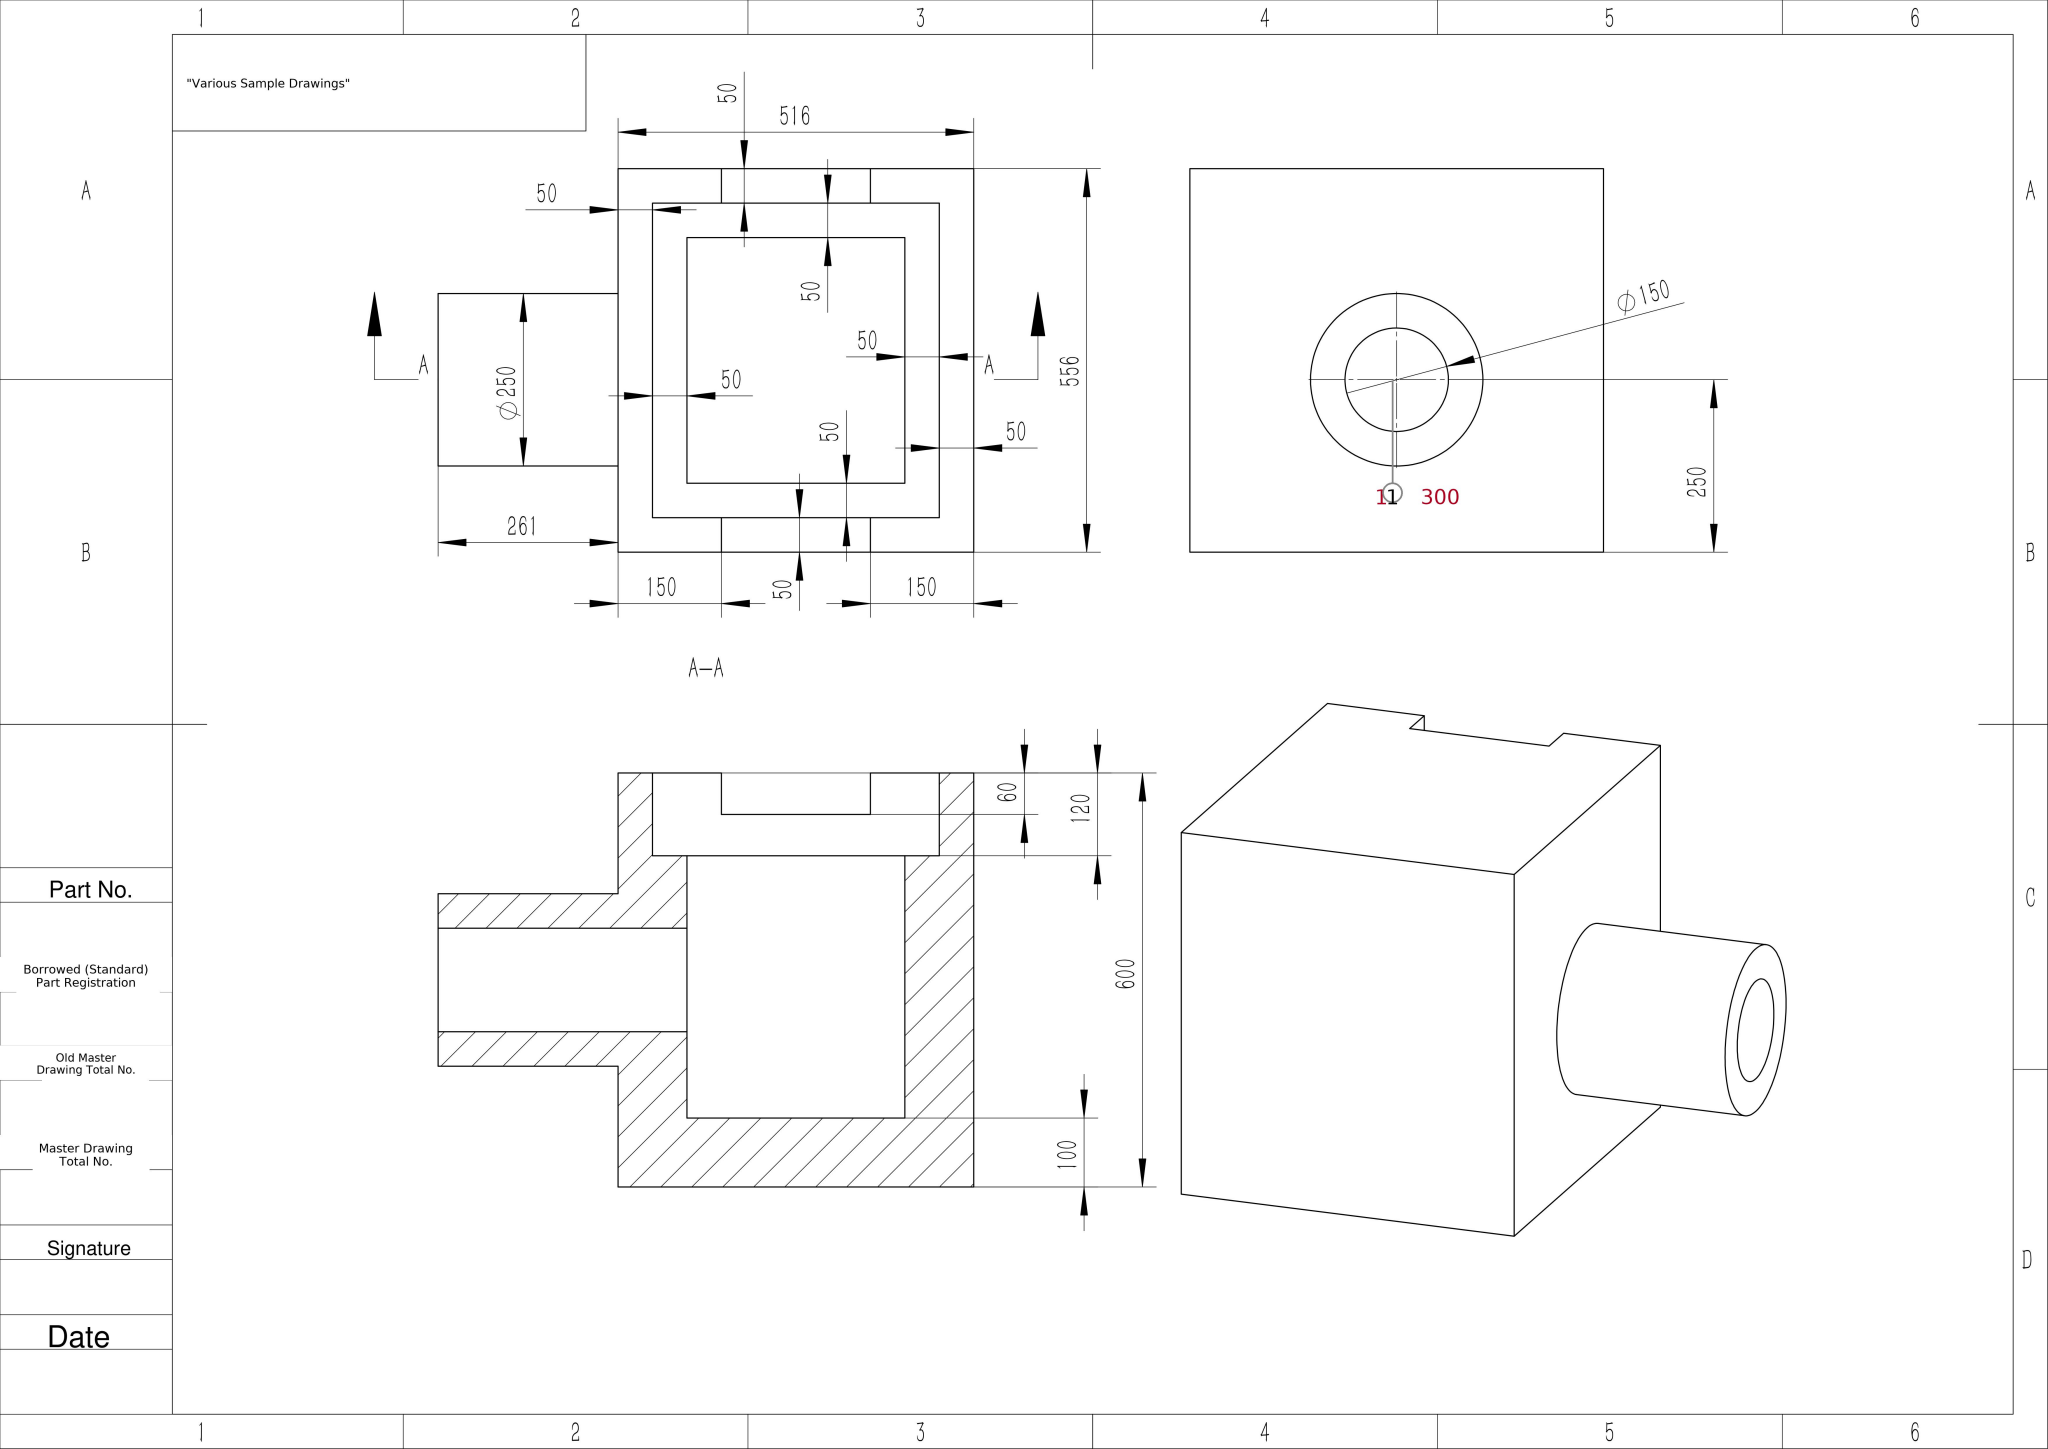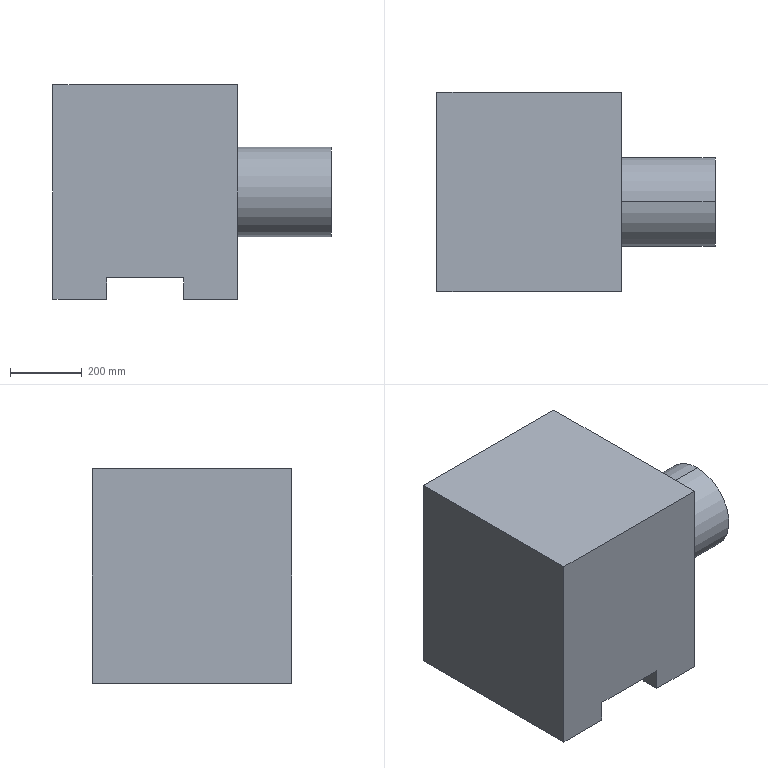Part | SolidWorks | mm | 1 solid | 28 faces | box 777 x 556 x 600 mm | volume 111762011 mm3 | plane 24 | cylinder 4 | commonest cylinder face diameters 150 x2 250 x2
build123d program:
from build123d import *

# Parameters (mm, degrees)
SKETCH1_W           = 516
SKETCH1_H           = 556
BOSS_EXTRUDE1_DEPTH = 600
SKETCH2_W           = 216
SKETCH2_H           = 597.069
CUT_EXTRUDE1_DEPTH  = 60
SKETCH3_W           = 416
SKETCH3_H           = 456
CUT_EXTRUDE2_DEPTH  = 120
SKETCH4_W           = 316
SKETCH4_H           = 356
CUT_EXTRUDE3_DEPTH  = 380
SKETCH6_R           = 125
SKETCH6_R_2         = 75
BOSS_EXTRUDE2_DEPTH = 261
CUT_EXTRUDE4_START  = -193
SKETCH7_R           = 75
CUT_EXTRUDE4_DEPTH  = 193


with BuildPart() as part:
    # Sketch1 → Boss-Extrude1 (new body)
    with BuildSketch(Plane.XY):
        Rectangle(SKETCH1_W, SKETCH1_H)
    extrude(amount=BOSS_EXTRUDE1_DEPTH)

    # Sketch2 → Cut-Extrude1 (cut)
    with BuildSketch(Plane(origin=(0, 0, 0), x_dir=(-1, 0, 0), z_dir=(0, 0, -1))):
        with Locations((0, -2.504)):
            Rectangle(SKETCH2_W, SKETCH2_H)
    extrude(amount=-CUT_EXTRUDE1_DEPTH, mode=Mode.SUBTRACT)

    # Sketch3 → Cut-Extrude2 (cut)
    with BuildSketch(Plane(origin=(0, 0, 0), x_dir=(-1, 0, 0), z_dir=(0, 0, -1))):
        Rectangle(SKETCH3_W, SKETCH3_H)
    extrude(amount=-CUT_EXTRUDE2_DEPTH, mode=Mode.SUBTRACT)

    # Sketch4 → Cut-Extrude3 (cut)
    with BuildSketch(Plane(origin=(0, 0, 120), x_dir=(-1, 0, 0), z_dir=(0, 0, -1))):
        Rectangle(SKETCH4_W, SKETCH4_H)
    extrude(amount=-CUT_EXTRUDE3_DEPTH, mode=Mode.SUBTRACT)

    # Sketch6 → Boss-Extrude2 (add)
    with BuildSketch(Plane(origin=(258, 0, 0), x_dir=(0, 0, -1), z_dir=(1, 0, 0))):
        with Locations((-300, -28)):
            Circle(SKETCH6_R)
        with Locations((-300, -28)):
            Circle(SKETCH6_R_2, mode=Mode.SUBTRACT)
    extrude(amount=BOSS_EXTRUDE2_DEPTH)

    # Sketch7 → Cut-Extrude4 (cut)
    with BuildSketch(Plane(origin=(258, 0, 0), x_dir=(0, 0, -1), z_dir=(1, 0, 0)).offset(CUT_EXTRUDE4_START)):
        with Locations((-300, -28)):
            Circle(SKETCH7_R)
    extrude(amount=CUT_EXTRUDE4_DEPTH, mode=Mode.SUBTRACT)


solid = part.part
STEP:
#1=CARTESIAN_POINT('',(519.,-28.,375.));
#2=VERTEX_POINT('',#1);
#3=CARTESIAN_POINT('',(519.,-28.,225.));
#4=VERTEX_POINT('',#3);
#5=CARTESIAN_POINT('',(519.,-28.,300.));
#6=DIRECTION('',(1.,0.,0.));
#7=DIRECTION('',(0.,0.,-1.));
#8=AXIS2_PLACEMENT_3D('',#5,#6,#7);
#9=CIRCLE('',#8,75.);
#10=EDGE_CURVE('',#2,#4,#9,.T.);
#11=ORIENTED_EDGE('',*,*,#10,.T.);
#12=CARTESIAN_POINT('',(158.,-28.,225.));
#13=VERTEX_POINT('',#12);
#14=CARTESIAN_POINT('',(519.,-28.,225.));
#15=DIRECTION('',(-1.,0.,0.));
#16=VECTOR('',#15,1000.);
#17=LINE('',#14,#16);
#18=EDGE_CURVE('',#4,#13,#17,.T.);
#19=ORIENTED_EDGE('',*,*,#18,.T.);
#20=CARTESIAN_POINT('',(158.,-28.,375.));
#21=VERTEX_POINT('',#20);
#22=CARTESIAN_POINT('',(158.,-28.,300.));
#23=DIRECTION('',(1.,0.,0.));
#24=DIRECTION('',(0.,0.,-1.));
#25=AXIS2_PLACEMENT_3D('',#22,#23,#24);
#26=CIRCLE('',#25,75.);
#27=EDGE_CURVE('',#21,#13,#26,.T.);
#28=ORIENTED_EDGE('',*,*,#27,.F.);
#29=CARTESIAN_POINT('',(519.,-28.,375.));
#30=DIRECTION('',(-1.,0.,0.));
#31=VECTOR('',#30,1000.);
#32=LINE('',#29,#31);
#33=EDGE_CURVE('',#2,#21,#32,.T.);
#34=ORIENTED_EDGE('',*,*,#33,.F.);
#35=EDGE_LOOP('',(#11,#19,#28,#34));
#36=FACE_OUTER_BOUND('',#35,.T.);
#37=CARTESIAN_POINT('',(519.,-28.,300.));
#38=DIRECTION('',(-1.,0.,0.));
#39=DIRECTION('',(0.,0.,1.));
#40=AXIS2_PLACEMENT_3D('',#37,#38,#39);
#41=CYLINDRICAL_SURFACE('',#40,75.);
#42=ADVANCED_FACE('',(#36),#41,.F.);
#43=CARTESIAN_POINT('',(519.,-28.,175.));
#44=VERTEX_POINT('',#43);
#45=CARTESIAN_POINT('',(519.,-28.,425.));
#46=VERTEX_POINT('',#45);
#47=CARTESIAN_POINT('',(519.,-28.,300.));
#48=DIRECTION('',(1.,0.,0.));
#49=DIRECTION('',(0.,0.,-1.));
#50=AXIS2_PLACEMENT_3D('',#47,#48,#49);
#51=CIRCLE('',#50,125.);
#52=EDGE_CURVE('',#44,#46,#51,.T.);
#53=ORIENTED_EDGE('',*,*,#52,.F.);
#54=CARTESIAN_POINT('',(258.,-28.,175.));
#55=VERTEX_POINT('',#54);
#56=CARTESIAN_POINT('',(519.,-28.,175.));
#57=DIRECTION('',(-1.,0.,0.));
#58=VECTOR('',#57,1000.);
#59=LINE('',#56,#58);
#60=EDGE_CURVE('',#44,#55,#59,.T.);
#61=ORIENTED_EDGE('',*,*,#60,.T.);
#62=CARTESIAN_POINT('',(258.,-28.,425.));
#63=VERTEX_POINT('',#62);
#64=CARTESIAN_POINT('',(258.,-28.,300.));
#65=DIRECTION('',(1.,0.,0.));
#66=DIRECTION('',(0.,0.,-1.));
#67=AXIS2_PLACEMENT_3D('',#64,#65,#66);
#68=CIRCLE('',#67,125.);
#69=EDGE_CURVE('',#55,#63,#68,.T.);
#70=ORIENTED_EDGE('',*,*,#69,.T.);
#71=CARTESIAN_POINT('',(519.,-28.,425.));
#72=DIRECTION('',(-1.,0.,0.));
#73=VECTOR('',#72,1000.);
#74=LINE('',#71,#73);
#75=EDGE_CURVE('',#46,#63,#74,.T.);
#76=ORIENTED_EDGE('',*,*,#75,.F.);
#77=EDGE_LOOP('',(#53,#61,#70,#76));
#78=FACE_OUTER_BOUND('',#77,.T.);
#79=CARTESIAN_POINT('',(519.,-28.,300.));
#80=DIRECTION('',(-1.,0.,0.));
#81=DIRECTION('',(0.,0.,1.));
#82=AXIS2_PLACEMENT_3D('',#79,#80,#81);
#83=CYLINDRICAL_SURFACE('',#82,125.);
#84=ADVANCED_FACE('',(#78),#83,.T.);
#85=CARTESIAN_POINT('',(-108.,228.,60.));
#86=VERTEX_POINT('',#85);
#87=CARTESIAN_POINT('',(108.,228.,60.));
#88=VERTEX_POINT('',#87);
#89=CARTESIAN_POINT('',(0.,228.,60.));
#90=DIRECTION('',(1.,0.,0.));
#91=VECTOR('',#90,1000.);
#92=LINE('',#89,#91);
#93=EDGE_CURVE('',#86,#88,#92,.T.);
#94=ORIENTED_EDGE('',*,*,#93,.F.);
#95=CARTESIAN_POINT('',(-108.,278.,60.));
#96=VERTEX_POINT('',#95);
#97=CARTESIAN_POINT('',(-108.,296.03,60.));
#98=DIRECTION('',(-0.,1.,0.));
#99=VECTOR('',#98,1000.);
#100=LINE('',#97,#99);
#101=EDGE_CURVE('',#86,#96,#100,.T.);
#102=ORIENTED_EDGE('',*,*,#101,.T.);
#103=CARTESIAN_POINT('',(108.,278.,60.));
#104=VERTEX_POINT('',#103);
#105=CARTESIAN_POINT('',(258.,278.,60.));
#106=DIRECTION('',(1.,0.,0.));
#107=VECTOR('',#106,1000.);
#108=LINE('',#105,#107);
#109=EDGE_CURVE('',#96,#104,#108,.T.);
#110=ORIENTED_EDGE('',*,*,#109,.T.);
#111=CARTESIAN_POINT('',(108.,296.03,60.));
#112=DIRECTION('',(-0.,-1.,0.));
#113=VECTOR('',#112,1000.);
#114=LINE('',#111,#113);
#115=EDGE_CURVE('',#104,#88,#114,.T.);
#116=ORIENTED_EDGE('',*,*,#115,.T.);
#117=EDGE_LOOP('',(#94,#102,#110,#116));
#118=FACE_OUTER_BOUND('',#117,.T.);
#119=CARTESIAN_POINT('',(0.,0.,60.));
#120=DIRECTION('',(0.,0.,-1.));
#121=DIRECTION('',(-1.,0.,0.));
#122=AXIS2_PLACEMENT_3D('',#119,#120,#121);
#123=PLANE('',#122);
#124=ADVANCED_FACE('',(#118),#123,.T.);
#125=CARTESIAN_POINT('',(108.,228.,0.));
#126=VERTEX_POINT('',#125);
#127=CARTESIAN_POINT('',(108.,278.,0.));
#128=VERTEX_POINT('',#127);
#129=CARTESIAN_POINT('',(108.,-0.,0.));
#130=DIRECTION('',(0.,1.,0.));
#131=VECTOR('',#130,1000.);
#132=LINE('',#129,#131);
#133=EDGE_CURVE('',#126,#128,#132,.T.);
#134=ORIENTED_EDGE('',*,*,#133,.F.);
#135=CARTESIAN_POINT('',(108.,228.,60.));
#136=DIRECTION('',(0.,0.,1.));
#137=VECTOR('',#136,1000.);
#138=LINE('',#135,#137);
#139=EDGE_CURVE('',#126,#88,#138,.T.);
#140=ORIENTED_EDGE('',*,*,#139,.T.);
#141=ORIENTED_EDGE('',*,*,#115,.F.);
#142=CARTESIAN_POINT('',(108.,278.,600.));
#143=DIRECTION('',(0.,0.,1.));
#144=VECTOR('',#143,1000.);
#145=LINE('',#142,#144);
#146=EDGE_CURVE('',#128,#104,#145,.T.);
#147=ORIENTED_EDGE('',*,*,#146,.F.);
#148=EDGE_LOOP('',(#134,#140,#141,#147));
#149=FACE_OUTER_BOUND('',#148,.T.);
#150=CARTESIAN_POINT('',(108.,296.03,60.));
#151=DIRECTION('',(1.,-0.,0.));
#152=DIRECTION('',(0.,1.,0.));
#153=AXIS2_PLACEMENT_3D('',#150,#151,#152);
#154=PLANE('',#153);
#155=ADVANCED_FACE('',(#149),#154,.F.);
#156=ORIENTED_EDGE('',*,*,#101,.F.);
#157=CARTESIAN_POINT('',(-108.,228.,0.));
#158=VERTEX_POINT('',#157);
#159=CARTESIAN_POINT('',(-108.,228.,60.));
#160=DIRECTION('',(0.,0.,-1.));
#161=VECTOR('',#160,1000.);
#162=LINE('',#159,#161);
#163=EDGE_CURVE('',#86,#158,#162,.T.);
#164=ORIENTED_EDGE('',*,*,#163,.T.);
#165=CARTESIAN_POINT('',(-108.,278.,0.));
#166=VERTEX_POINT('',#165);
#167=CARTESIAN_POINT('',(-108.,-0.,0.));
#168=DIRECTION('',(0.,-1.,0.));
#169=VECTOR('',#168,1000.);
#170=LINE('',#167,#169);
#171=EDGE_CURVE('',#166,#158,#170,.T.);
#172=ORIENTED_EDGE('',*,*,#171,.F.);
#173=CARTESIAN_POINT('',(-108.,278.,600.));
#174=DIRECTION('',(0.,0.,-1.));
#175=VECTOR('',#174,1000.);
#176=LINE('',#173,#175);
#177=EDGE_CURVE('',#96,#166,#176,.T.);
#178=ORIENTED_EDGE('',*,*,#177,.F.);
#179=EDGE_LOOP('',(#156,#164,#172,#178));
#180=FACE_OUTER_BOUND('',#179,.T.);
#181=CARTESIAN_POINT('',(-108.,296.03,60.));
#182=DIRECTION('',(-1.,-0.,0.));
#183=DIRECTION('',(0.,-1.,0.));
#184=AXIS2_PLACEMENT_3D('',#181,#182,#183);
#185=PLANE('',#184);
#186=ADVANCED_FACE('',(#180),#185,.F.);
#187=CARTESIAN_POINT('',(208.,228.,0.));
#188=VERTEX_POINT('',#187);
#189=CARTESIAN_POINT('',(208.,-228.,0.));
#190=VERTEX_POINT('',#189);
#191=CARTESIAN_POINT('',(208.,-228.,0.));
#192=DIRECTION('',(0.,-1.,0.));
#193=VECTOR('',#192,1000.);
#194=LINE('',#191,#193);
#195=EDGE_CURVE('',#188,#190,#194,.T.);
#196=ORIENTED_EDGE('',*,*,#195,.F.);
#197=CARTESIAN_POINT('',(-208.,228.,0.));
#198=DIRECTION('',(1.,0.,0.));
#199=VECTOR('',#198,1000.);
#200=LINE('',#197,#199);
#201=EDGE_CURVE('',#126,#188,#200,.T.);
#202=ORIENTED_EDGE('',*,*,#201,.F.);
#203=ORIENTED_EDGE('',*,*,#133,.T.);
#204=CARTESIAN_POINT('',(258.,278.,0.));
#205=VERTEX_POINT('',#204);
#206=CARTESIAN_POINT('',(258.,278.,0.));
#207=DIRECTION('',(-1.,-0.,0.));
#208=VECTOR('',#207,1000.);
#209=LINE('',#206,#208);
#210=EDGE_CURVE('',#205,#128,#209,.T.);
#211=ORIENTED_EDGE('',*,*,#210,.F.);
#212=CARTESIAN_POINT('',(258.,-278.,0.));
#213=VERTEX_POINT('',#212);
#214=CARTESIAN_POINT('',(258.,-278.,0.));
#215=DIRECTION('',(0.,1.,0.));
#216=VECTOR('',#215,1000.);
#217=LINE('',#214,#216);
#218=EDGE_CURVE('',#213,#205,#217,.T.);
#219=ORIENTED_EDGE('',*,*,#218,.F.);
#220=CARTESIAN_POINT('',(108.,-278.,0.));
#221=VERTEX_POINT('',#220);
#222=CARTESIAN_POINT('',(258.,-278.,0.));
#223=DIRECTION('',(1.,0.,0.));
#224=VECTOR('',#223,1000.);
#225=LINE('',#222,#224);
#226=EDGE_CURVE('',#221,#213,#225,.T.);
#227=ORIENTED_EDGE('',*,*,#226,.F.);
#228=CARTESIAN_POINT('',(108.,-228.,0.));
#229=VERTEX_POINT('',#228);
#230=CARTESIAN_POINT('',(108.,-0.,0.));
#231=DIRECTION('',(0.,1.,0.));
#232=VECTOR('',#231,1000.);
#233=LINE('',#230,#232);
#234=EDGE_CURVE('',#221,#229,#233,.T.);
#235=ORIENTED_EDGE('',*,*,#234,.T.);
#236=CARTESIAN_POINT('',(-208.,-228.,0.));
#237=DIRECTION('',(-1.,0.,0.));
#238=VECTOR('',#237,1000.);
#239=LINE('',#236,#238);
#240=EDGE_CURVE('',#190,#229,#239,.T.);
#241=ORIENTED_EDGE('',*,*,#240,.F.);
#242=EDGE_LOOP('',(#196,#202,#203,#211,#219,#227,#235,#241));
#243=FACE_OUTER_BOUND('',#242,.T.);
#244=CARTESIAN_POINT('',(0.,0.,0.));
#245=DIRECTION('',(0.,0.,1.));
#246=DIRECTION('',(1.,0.,0.));
#247=AXIS2_PLACEMENT_3D('',#244,#245,#246);
#248=PLANE('',#247);
#249=ADVANCED_FACE('',(#243),#248,.F.);
#250=CARTESIAN_POINT('',(-258.,278.,0.));
#251=VERTEX_POINT('',#250);
#252=CARTESIAN_POINT('',(-258.,-278.,0.));
#253=VERTEX_POINT('',#252);
#254=CARTESIAN_POINT('',(-258.,-278.,0.));
#255=DIRECTION('',(0.,-1.,0.));
#256=VECTOR('',#255,1000.);
#257=LINE('',#254,#256);
#258=EDGE_CURVE('',#251,#253,#257,.T.);
#259=ORIENTED_EDGE('',*,*,#258,.T.);
#260=CARTESIAN_POINT('',(-258.,-278.,600.));
#261=VERTEX_POINT('',#260);
#262=CARTESIAN_POINT('',(-258.,-278.,600.));
#263=DIRECTION('',(0.,0.,-1.));
#264=VECTOR('',#263,1000.);
#265=LINE('',#262,#264);
#266=EDGE_CURVE('',#261,#253,#265,.T.);
#267=ORIENTED_EDGE('',*,*,#266,.F.);
#268=CARTESIAN_POINT('',(-258.,278.,600.));
#269=VERTEX_POINT('',#268);
#270=CARTESIAN_POINT('',(-258.,-278.,600.));
#271=DIRECTION('',(0.,-1.,0.));
#272=VECTOR('',#271,1000.);
#273=LINE('',#270,#272);
#274=EDGE_CURVE('',#269,#261,#273,.T.);
#275=ORIENTED_EDGE('',*,*,#274,.F.);
#276=CARTESIAN_POINT('',(-258.,278.,600.));
#277=DIRECTION('',(0.,0.,-1.));
#278=VECTOR('',#277,1000.);
#279=LINE('',#276,#278);
#280=EDGE_CURVE('',#269,#251,#279,.T.);
#281=ORIENTED_EDGE('',*,*,#280,.T.);
#282=EDGE_LOOP('',(#259,#267,#275,#281));
#283=FACE_OUTER_BOUND('',#282,.T.);
#284=CARTESIAN_POINT('',(-258.,-278.,600.));
#285=DIRECTION('',(1.,0.,0.));
#286=DIRECTION('',(0.,0.,-1.));
#287=AXIS2_PLACEMENT_3D('',#284,#285,#286);
#288=PLANE('',#287);
#289=ADVANCED_FACE('',(#283),#288,.F.);
#290=CARTESIAN_POINT('',(108.,-278.,60.));
#291=VERTEX_POINT('',#290);
#292=CARTESIAN_POINT('',(-108.,-278.,60.));
#293=VERTEX_POINT('',#292);
#294=CARTESIAN_POINT('',(258.,-278.,60.));
#295=DIRECTION('',(-1.,-0.,0.));
#296=VECTOR('',#295,1000.);
#297=LINE('',#294,#296);
#298=EDGE_CURVE('',#291,#293,#297,.T.);
#299=ORIENTED_EDGE('',*,*,#298,.F.);
#300=CARTESIAN_POINT('',(108.,-278.,600.));
#301=DIRECTION('',(0.,0.,-1.));
#302=VECTOR('',#301,1000.);
#303=LINE('',#300,#302);
#304=EDGE_CURVE('',#291,#221,#303,.T.);
#305=ORIENTED_EDGE('',*,*,#304,.T.);
#306=ORIENTED_EDGE('',*,*,#226,.T.);
#307=CARTESIAN_POINT('',(258.,-278.,600.));
#308=VERTEX_POINT('',#307);
#309=CARTESIAN_POINT('',(258.,-278.,600.));
#310=DIRECTION('',(0.,0.,-1.));
#311=VECTOR('',#310,1000.);
#312=LINE('',#309,#311);
#313=EDGE_CURVE('',#308,#213,#312,.T.);
#314=ORIENTED_EDGE('',*,*,#313,.F.);
#315=CARTESIAN_POINT('',(258.,-278.,600.));
#316=DIRECTION('',(1.,0.,0.));
#317=VECTOR('',#316,1000.);
#318=LINE('',#315,#317);
#319=EDGE_CURVE('',#261,#308,#318,.T.);
#320=ORIENTED_EDGE('',*,*,#319,.F.);
#321=ORIENTED_EDGE('',*,*,#266,.T.);
#322=CARTESIAN_POINT('',(-108.,-278.,0.));
#323=VERTEX_POINT('',#322);
#324=CARTESIAN_POINT('',(258.,-278.,0.));
#325=DIRECTION('',(1.,0.,0.));
#326=VECTOR('',#325,1000.);
#327=LINE('',#324,#326);
#328=EDGE_CURVE('',#253,#323,#327,.T.);
#329=ORIENTED_EDGE('',*,*,#328,.T.);
#330=CARTESIAN_POINT('',(-108.,-278.,600.));
#331=DIRECTION('',(0.,0.,1.));
#332=VECTOR('',#331,1000.);
#333=LINE('',#330,#332);
#334=EDGE_CURVE('',#323,#293,#333,.T.);
#335=ORIENTED_EDGE('',*,*,#334,.T.);
#336=EDGE_LOOP('',(#299,#305,#306,#314,#320,#321,#329,#335));
#337=FACE_OUTER_BOUND('',#336,.T.);
#338=CARTESIAN_POINT('',(258.,-278.,600.));
#339=DIRECTION('',(-0.,1.,0.));
#340=DIRECTION('',(-1.,-0.,0.));
#341=AXIS2_PLACEMENT_3D('',#338,#339,#340);
#342=PLANE('',#341);
#343=ADVANCED_FACE('',(#337),#342,.F.);
#344=CARTESIAN_POINT('',(258.,-28.,300.));
#345=DIRECTION('',(1.,0.,0.));
#346=DIRECTION('',(0.,0.,-1.));
#347=AXIS2_PLACEMENT_3D('',#344,#345,#346);
#348=CIRCLE('',#347,125.);
#349=EDGE_CURVE('',#63,#55,#348,.T.);
#350=ORIENTED_EDGE('',*,*,#349,.F.);
#351=ORIENTED_EDGE('',*,*,#69,.F.);
#352=EDGE_LOOP('',(#350,#351));
#353=FACE_BOUND('',#352,.T.);
#354=ORIENTED_EDGE('',*,*,#218,.T.);
#355=CARTESIAN_POINT('',(258.,278.,600.));
#356=VERTEX_POINT('',#355);
#357=CARTESIAN_POINT('',(258.,278.,600.));
#358=DIRECTION('',(0.,0.,-1.));
#359=VECTOR('',#358,1000.);
#360=LINE('',#357,#359);
#361=EDGE_CURVE('',#356,#205,#360,.T.);
#362=ORIENTED_EDGE('',*,*,#361,.F.);
#363=CARTESIAN_POINT('',(258.,-278.,600.));
#364=DIRECTION('',(0.,1.,0.));
#365=VECTOR('',#364,1000.);
#366=LINE('',#363,#365);
#367=EDGE_CURVE('',#308,#356,#366,.T.);
#368=ORIENTED_EDGE('',*,*,#367,.F.);
#369=ORIENTED_EDGE('',*,*,#313,.T.);
#370=EDGE_LOOP('',(#354,#362,#368,#369));
#371=FACE_OUTER_BOUND('',#370,.T.);
#372=CARTESIAN_POINT('',(258.,-278.,600.));
#373=DIRECTION('',(-1.,0.,0.));
#374=DIRECTION('',(0.,0.,1.));
#375=AXIS2_PLACEMENT_3D('',#372,#373,#374);
#376=PLANE('',#375);
#377=ADVANCED_FACE('',(#353,#371),#376,.F.);
#378=ORIENTED_EDGE('',*,*,#210,.T.);
#379=ORIENTED_EDGE('',*,*,#146,.T.);
#380=ORIENTED_EDGE('',*,*,#109,.F.);
#381=ORIENTED_EDGE('',*,*,#177,.T.);
#382=CARTESIAN_POINT('',(258.,278.,0.));
#383=DIRECTION('',(-1.,-0.,0.));
#384=VECTOR('',#383,1000.);
#385=LINE('',#382,#384);
#386=EDGE_CURVE('',#166,#251,#385,.T.);
#387=ORIENTED_EDGE('',*,*,#386,.T.);
#388=ORIENTED_EDGE('',*,*,#280,.F.);
#389=CARTESIAN_POINT('',(258.,278.,600.));
#390=DIRECTION('',(-1.,-0.,0.));
#391=VECTOR('',#390,1000.);
#392=LINE('',#389,#391);
#393=EDGE_CURVE('',#356,#269,#392,.T.);
#394=ORIENTED_EDGE('',*,*,#393,.F.);
#395=ORIENTED_EDGE('',*,*,#361,.T.);
#396=EDGE_LOOP('',(#378,#379,#380,#381,#387,#388,#394,#395));
#397=FACE_OUTER_BOUND('',#396,.T.);
#398=CARTESIAN_POINT('',(258.,278.,600.));
#399=DIRECTION('',(0.,-1.,0.));
#400=DIRECTION('',(1.,0.,0.));
#401=AXIS2_PLACEMENT_3D('',#398,#399,#400);
#402=PLANE('',#401);
#403=ADVANCED_FACE('',(#397),#402,.F.);
#404=ORIENTED_EDGE('',*,*,#274,.T.);
#405=ORIENTED_EDGE('',*,*,#319,.T.);
#406=ORIENTED_EDGE('',*,*,#367,.T.);
#407=ORIENTED_EDGE('',*,*,#393,.T.);
#408=EDGE_LOOP('',(#404,#405,#406,#407));
#409=FACE_OUTER_BOUND('',#408,.T.);
#410=CARTESIAN_POINT('',(0.,0.,600.));
#411=DIRECTION('',(0.,0.,1.));
#412=DIRECTION('',(1.,0.,0.));
#413=AXIS2_PLACEMENT_3D('',#410,#411,#412);
#414=PLANE('',#413);
#415=ADVANCED_FACE('',(#409),#414,.T.);
#416=ORIENTED_EDGE('',*,*,#171,.T.);
#417=CARTESIAN_POINT('',(-208.,228.,0.));
#418=VERTEX_POINT('',#417);
#419=CARTESIAN_POINT('',(-208.,228.,0.));
#420=DIRECTION('',(1.,0.,0.));
#421=VECTOR('',#420,1000.);
#422=LINE('',#419,#421);
#423=EDGE_CURVE('',#418,#158,#422,.T.);
#424=ORIENTED_EDGE('',*,*,#423,.F.);
#425=CARTESIAN_POINT('',(-208.,-228.,0.));
#426=VERTEX_POINT('',#425);
#427=CARTESIAN_POINT('',(-208.,-228.,0.));
#428=DIRECTION('',(0.,1.,0.));
#429=VECTOR('',#428,1000.);
#430=LINE('',#427,#429);
#431=EDGE_CURVE('',#426,#418,#430,.T.);
#432=ORIENTED_EDGE('',*,*,#431,.F.);
#433=CARTESIAN_POINT('',(-108.,-228.,0.));
#434=VERTEX_POINT('',#433);
#435=CARTESIAN_POINT('',(-208.,-228.,0.));
#436=DIRECTION('',(-1.,0.,0.));
#437=VECTOR('',#436,1000.);
#438=LINE('',#435,#437);
#439=EDGE_CURVE('',#434,#426,#438,.T.);
#440=ORIENTED_EDGE('',*,*,#439,.F.);
#441=CARTESIAN_POINT('',(-108.,-0.,0.));
#442=DIRECTION('',(0.,-1.,0.));
#443=VECTOR('',#442,1000.);
#444=LINE('',#441,#443);
#445=EDGE_CURVE('',#434,#323,#444,.T.);
#446=ORIENTED_EDGE('',*,*,#445,.T.);
#447=ORIENTED_EDGE('',*,*,#328,.F.);
#448=ORIENTED_EDGE('',*,*,#258,.F.);
#449=ORIENTED_EDGE('',*,*,#386,.F.);
#450=EDGE_LOOP('',(#416,#424,#432,#440,#446,#447,#448,#449));
#451=FACE_OUTER_BOUND('',#450,.T.);
#452=CARTESIAN_POINT('',(0.,0.,0.));
#453=DIRECTION('',(0.,0.,1.));
#454=DIRECTION('',(1.,0.,0.));
#455=AXIS2_PLACEMENT_3D('',#452,#453,#454);
#456=PLANE('',#455);
#457=ADVANCED_FACE('',(#451),#456,.F.);
#458=CARTESIAN_POINT('',(108.,-228.,60.));
#459=VERTEX_POINT('',#458);
#460=CARTESIAN_POINT('',(-108.,-228.,60.));
#461=VERTEX_POINT('',#460);
#462=CARTESIAN_POINT('',(0.,-228.,60.));
#463=DIRECTION('',(-1.,0.,0.));
#464=VECTOR('',#463,1000.);
#465=LINE('',#462,#464);
#466=EDGE_CURVE('',#459,#461,#465,.T.);
#467=ORIENTED_EDGE('',*,*,#466,.F.);
#468=CARTESIAN_POINT('',(108.,296.03,60.));
#469=DIRECTION('',(-0.,-1.,0.));
#470=VECTOR('',#469,1000.);
#471=LINE('',#468,#470);
#472=EDGE_CURVE('',#459,#291,#471,.T.);
#473=ORIENTED_EDGE('',*,*,#472,.T.);
#474=ORIENTED_EDGE('',*,*,#298,.T.);
#475=CARTESIAN_POINT('',(-108.,296.03,60.));
#476=DIRECTION('',(-0.,1.,0.));
#477=VECTOR('',#476,1000.);
#478=LINE('',#475,#477);
#479=EDGE_CURVE('',#293,#461,#478,.T.);
#480=ORIENTED_EDGE('',*,*,#479,.T.);
#481=EDGE_LOOP('',(#467,#473,#474,#480));
#482=FACE_OUTER_BOUND('',#481,.T.);
#483=CARTESIAN_POINT('',(0.,0.,60.));
#484=DIRECTION('',(0.,0.,-1.));
#485=DIRECTION('',(-1.,0.,0.));
#486=AXIS2_PLACEMENT_3D('',#483,#484,#485);
#487=PLANE('',#486);
#488=ADVANCED_FACE('',(#482),#487,.T.);
#489=ORIENTED_EDGE('',*,*,#472,.F.);
#490=CARTESIAN_POINT('',(108.,-228.,60.));
#491=DIRECTION('',(0.,0.,-1.));
#492=VECTOR('',#491,1000.);
#493=LINE('',#490,#492);
#494=EDGE_CURVE('',#459,#229,#493,.T.);
#495=ORIENTED_EDGE('',*,*,#494,.T.);
#496=ORIENTED_EDGE('',*,*,#234,.F.);
#497=ORIENTED_EDGE('',*,*,#304,.F.);
#498=EDGE_LOOP('',(#489,#495,#496,#497));
#499=FACE_OUTER_BOUND('',#498,.T.);
#500=CARTESIAN_POINT('',(108.,296.03,60.));
#501=DIRECTION('',(1.,-0.,0.));
#502=DIRECTION('',(0.,1.,0.));
#503=AXIS2_PLACEMENT_3D('',#500,#501,#502);
#504=PLANE('',#503);
#505=ADVANCED_FACE('',(#499),#504,.F.);
#506=ORIENTED_EDGE('',*,*,#445,.F.);
#507=CARTESIAN_POINT('',(-108.,-228.,60.));
#508=DIRECTION('',(0.,0.,1.));
#509=VECTOR('',#508,1000.);
#510=LINE('',#507,#509);
#511=EDGE_CURVE('',#434,#461,#510,.T.);
#512=ORIENTED_EDGE('',*,*,#511,.T.);
#513=ORIENTED_EDGE('',*,*,#479,.F.);
#514=ORIENTED_EDGE('',*,*,#334,.F.);
#515=EDGE_LOOP('',(#506,#512,#513,#514));
#516=FACE_OUTER_BOUND('',#515,.T.);
#517=CARTESIAN_POINT('',(-108.,296.03,60.));
#518=DIRECTION('',(-1.,-0.,0.));
#519=DIRECTION('',(0.,-1.,0.));
#520=AXIS2_PLACEMENT_3D('',#517,#518,#519);
#521=PLANE('',#520);
#522=ADVANCED_FACE('',(#516),#521,.F.);
#523=ORIENTED_EDGE('',*,*,#201,.T.);
#524=CARTESIAN_POINT('',(208.,228.,120.));
#525=VERTEX_POINT('',#524);
#526=CARTESIAN_POINT('',(208.,228.,120.));
#527=DIRECTION('',(0.,0.,-1.));
#528=VECTOR('',#527,1000.);
#529=LINE('',#526,#528);
#530=EDGE_CURVE('',#525,#188,#529,.T.);
#531=ORIENTED_EDGE('',*,*,#530,.F.);
#532=CARTESIAN_POINT('',(-208.,228.,120.));
#533=VERTEX_POINT('',#532);
#534=CARTESIAN_POINT('',(-208.,228.,120.));
#535=DIRECTION('',(1.,0.,0.));
#536=VECTOR('',#535,1000.);
#537=LINE('',#534,#536);
#538=EDGE_CURVE('',#533,#525,#537,.T.);
#539=ORIENTED_EDGE('',*,*,#538,.F.);
#540=CARTESIAN_POINT('',(-208.,228.,120.));
#541=DIRECTION('',(0.,0.,-1.));
#542=VECTOR('',#541,1000.);
#543=LINE('',#540,#542);
#544=EDGE_CURVE('',#533,#418,#543,.T.);
#545=ORIENTED_EDGE('',*,*,#544,.T.);
#546=ORIENTED_EDGE('',*,*,#423,.T.);
#547=ORIENTED_EDGE('',*,*,#163,.F.);
#548=ORIENTED_EDGE('',*,*,#93,.T.);
#549=ORIENTED_EDGE('',*,*,#139,.F.);
#550=EDGE_LOOP('',(#523,#531,#539,#545,#546,#547,#548,#549));
#551=FACE_OUTER_BOUND('',#550,.T.);
#552=CARTESIAN_POINT('',(-208.,228.,120.));
#553=DIRECTION('',(0.,1.,0.));
#554=DIRECTION('',(0.,0.,1.));
#555=AXIS2_PLACEMENT_3D('',#552,#553,#554);
#556=PLANE('',#555);
#557=ADVANCED_FACE('',(#551),#556,.F.);
#558=ORIENTED_EDGE('',*,*,#466,.T.);
#559=ORIENTED_EDGE('',*,*,#511,.F.);
#560=ORIENTED_EDGE('',*,*,#439,.T.);
#561=CARTESIAN_POINT('',(-208.,-228.,120.));
#562=VERTEX_POINT('',#561);
#563=CARTESIAN_POINT('',(-208.,-228.,120.));
#564=DIRECTION('',(0.,0.,-1.));
#565=VECTOR('',#564,1000.);
#566=LINE('',#563,#565);
#567=EDGE_CURVE('',#562,#426,#566,.T.);
#568=ORIENTED_EDGE('',*,*,#567,.F.);
#569=CARTESIAN_POINT('',(208.,-228.,120.));
#570=VERTEX_POINT('',#569);
#571=CARTESIAN_POINT('',(-208.,-228.,120.));
#572=DIRECTION('',(-1.,0.,0.));
#573=VECTOR('',#572,1000.);
#574=LINE('',#571,#573);
#575=EDGE_CURVE('',#570,#562,#574,.T.);
#576=ORIENTED_EDGE('',*,*,#575,.F.);
#577=CARTESIAN_POINT('',(208.,-228.,120.));
#578=DIRECTION('',(0.,0.,-1.));
#579=VECTOR('',#578,1000.);
#580=LINE('',#577,#579);
#581=EDGE_CURVE('',#570,#190,#580,.T.);
#582=ORIENTED_EDGE('',*,*,#581,.T.);
#583=ORIENTED_EDGE('',*,*,#240,.T.);
#584=ORIENTED_EDGE('',*,*,#494,.F.);
#585=EDGE_LOOP('',(#558,#559,#560,#568,#576,#582,#583,#584));
#586=FACE_OUTER_BOUND('',#585,.T.);
#587=CARTESIAN_POINT('',(-208.,-228.,120.));
#588=DIRECTION('',(0.,-1.,0.));
#589=DIRECTION('',(0.,0.,-1.));
#590=AXIS2_PLACEMENT_3D('',#587,#588,#589);
#591=PLANE('',#590);
#592=ADVANCED_FACE('',(#586),#591,.F.);
#593=ORIENTED_EDGE('',*,*,#195,.T.);
#594=ORIENTED_EDGE('',*,*,#581,.F.);
#595=CARTESIAN_POINT('',(208.,-228.,120.));
#596=DIRECTION('',(0.,-1.,0.));
#597=VECTOR('',#596,1000.);
#598=LINE('',#595,#597);
#599=EDGE_CURVE('',#525,#570,#598,.T.);
#600=ORIENTED_EDGE('',*,*,#599,.F.);
#601=ORIENTED_EDGE('',*,*,#530,.T.);
#602=EDGE_LOOP('',(#593,#594,#600,#601));
#603=FACE_OUTER_BOUND('',#602,.T.);
#604=CARTESIAN_POINT('',(208.,-228.,120.));
#605=DIRECTION('',(1.,0.,0.));
#606=DIRECTION('',(0.,0.,-1.));
#607=AXIS2_PLACEMENT_3D('',#604,#605,#606);
#608=PLANE('',#607);
#609=ADVANCED_FACE('',(#603),#608,.F.);
#610=ORIENTED_EDGE('',*,*,#431,.T.);
#611=ORIENTED_EDGE('',*,*,#544,.F.);
#612=CARTESIAN_POINT('',(-208.,-228.,120.));
#613=DIRECTION('',(0.,1.,0.));
#614=VECTOR('',#613,1000.);
#615=LINE('',#612,#614);
#616=EDGE_CURVE('',#562,#533,#615,.T.);
#617=ORIENTED_EDGE('',*,*,#616,.F.);
#618=ORIENTED_EDGE('',*,*,#567,.T.);
#619=EDGE_LOOP('',(#610,#611,#617,#618));
#620=FACE_OUTER_BOUND('',#619,.T.);
#621=CARTESIAN_POINT('',(-208.,-228.,120.));
#622=DIRECTION('',(-1.,0.,0.));
#623=DIRECTION('',(0.,0.,1.));
#624=AXIS2_PLACEMENT_3D('',#621,#622,#623);
#625=PLANE('',#624);
#626=ADVANCED_FACE('',(#620),#625,.F.);
#627=CARTESIAN_POINT('',(-158.,178.,120.));
#628=VERTEX_POINT('',#627);
#629=CARTESIAN_POINT('',(158.,178.,120.));
#630=VERTEX_POINT('',#629);
#631=CARTESIAN_POINT('',(-158.,178.,120.));
#632=DIRECTION('',(1.,0.,0.));
#633=VECTOR('',#632,1000.);
#634=LINE('',#631,#633);
#635=EDGE_CURVE('',#628,#630,#634,.T.);
#636=ORIENTED_EDGE('',*,*,#635,.F.);
#637=CARTESIAN_POINT('',(-158.,-178.,120.));
#638=VERTEX_POINT('',#637);
#639=CARTESIAN_POINT('',(-158.,-178.,120.));
#640=DIRECTION('',(0.,1.,0.));
#641=VECTOR('',#640,1000.);
#642=LINE('',#639,#641);
#643=EDGE_CURVE('',#638,#628,#642,.T.);
#644=ORIENTED_EDGE('',*,*,#643,.F.);
#645=CARTESIAN_POINT('',(158.,-178.,120.));
#646=VERTEX_POINT('',#645);
#647=CARTESIAN_POINT('',(158.,-178.,120.));
#648=DIRECTION('',(-1.,0.,0.));
#649=VECTOR('',#648,1000.);
#650=LINE('',#647,#649);
#651=EDGE_CURVE('',#646,#638,#650,.T.);
#652=ORIENTED_EDGE('',*,*,#651,.F.);
#653=CARTESIAN_POINT('',(158.,178.,120.));
#654=DIRECTION('',(0.,-1.,0.));
#655=VECTOR('',#654,1000.);
#656=LINE('',#653,#655);
#657=EDGE_CURVE('',#630,#646,#656,.T.);
#658=ORIENTED_EDGE('',*,*,#657,.F.);
#659=EDGE_LOOP('',(#636,#644,#652,#658));
#660=FACE_BOUND('',#659,.T.);
#661=ORIENTED_EDGE('',*,*,#599,.T.);
#662=ORIENTED_EDGE('',*,*,#575,.T.);
#663=ORIENTED_EDGE('',*,*,#616,.T.);
#664=ORIENTED_EDGE('',*,*,#538,.T.);
#665=EDGE_LOOP('',(#661,#662,#663,#664));
#666=FACE_OUTER_BOUND('',#665,.T.);
#667=CARTESIAN_POINT('',(0.,0.,120.));
#668=DIRECTION('',(0.,0.,-1.));
#669=DIRECTION('',(-1.,0.,0.));
#670=AXIS2_PLACEMENT_3D('',#667,#668,#669);
#671=PLANE('',#670);
#672=ADVANCED_FACE('',(#660,#666),#671,.T.);
#673=ORIENTED_EDGE('',*,*,#635,.T.);
#674=CARTESIAN_POINT('',(158.,178.,500.));
#675=VERTEX_POINT('',#674);
#676=CARTESIAN_POINT('',(158.,178.,500.));
#677=DIRECTION('',(0.,0.,-1.));
#678=VECTOR('',#677,1000.);
#679=LINE('',#676,#678);
#680=EDGE_CURVE('',#675,#630,#679,.T.);
#681=ORIENTED_EDGE('',*,*,#680,.F.);
#682=CARTESIAN_POINT('',(-158.,178.,500.));
#683=VERTEX_POINT('',#682);
#684=CARTESIAN_POINT('',(-158.,178.,500.));
#685=DIRECTION('',(1.,0.,0.));
#686=VECTOR('',#685,1000.);
#687=LINE('',#684,#686);
#688=EDGE_CURVE('',#683,#675,#687,.T.);
#689=ORIENTED_EDGE('',*,*,#688,.F.);
#690=CARTESIAN_POINT('',(-158.,178.,500.));
#691=DIRECTION('',(0.,0.,-1.));
#692=VECTOR('',#691,1000.);
#693=LINE('',#690,#692);
#694=EDGE_CURVE('',#683,#628,#693,.T.);
#695=ORIENTED_EDGE('',*,*,#694,.T.);
#696=EDGE_LOOP('',(#673,#681,#689,#695));
#697=FACE_OUTER_BOUND('',#696,.T.);
#698=CARTESIAN_POINT('',(-158.,178.,500.));
#699=DIRECTION('',(0.,1.,0.));
#700=DIRECTION('',(0.,0.,1.));
#701=AXIS2_PLACEMENT_3D('',#698,#699,#700);
#702=PLANE('',#701);
#703=ADVANCED_FACE('',(#697),#702,.F.);
#704=ORIENTED_EDGE('',*,*,#643,.T.);
#705=ORIENTED_EDGE('',*,*,#694,.F.);
#706=CARTESIAN_POINT('',(-158.,-178.,500.));
#707=VERTEX_POINT('',#706);
#708=CARTESIAN_POINT('',(-158.,-178.,500.));
#709=DIRECTION('',(0.,1.,0.));
#710=VECTOR('',#709,1000.);
#711=LINE('',#708,#710);
#712=EDGE_CURVE('',#707,#683,#711,.T.);
#713=ORIENTED_EDGE('',*,*,#712,.F.);
#714=CARTESIAN_POINT('',(-158.,-178.,500.));
#715=DIRECTION('',(0.,0.,-1.));
#716=VECTOR('',#715,1000.);
#717=LINE('',#714,#716);
#718=EDGE_CURVE('',#707,#638,#717,.T.);
#719=ORIENTED_EDGE('',*,*,#718,.T.);
#720=EDGE_LOOP('',(#704,#705,#713,#719));
#721=FACE_OUTER_BOUND('',#720,.T.);
#722=CARTESIAN_POINT('',(-158.,-178.,500.));
#723=DIRECTION('',(-1.,0.,0.));
#724=DIRECTION('',(0.,0.,1.));
#725=AXIS2_PLACEMENT_3D('',#722,#723,#724);
#726=PLANE('',#725);
#727=ADVANCED_FACE('',(#721),#726,.F.);
#728=ORIENTED_EDGE('',*,*,#651,.T.);
#729=ORIENTED_EDGE('',*,*,#718,.F.);
#730=CARTESIAN_POINT('',(158.,-178.,500.));
#731=VERTEX_POINT('',#730);
#732=CARTESIAN_POINT('',(158.,-178.,500.));
#733=DIRECTION('',(-1.,0.,0.));
#734=VECTOR('',#733,1000.);
#735=LINE('',#732,#734);
#736=EDGE_CURVE('',#731,#707,#735,.T.);
#737=ORIENTED_EDGE('',*,*,#736,.F.);
#738=CARTESIAN_POINT('',(158.,-178.,500.));
#739=DIRECTION('',(0.,0.,-1.));
#740=VECTOR('',#739,1000.);
#741=LINE('',#738,#740);
#742=EDGE_CURVE('',#731,#646,#741,.T.);
#743=ORIENTED_EDGE('',*,*,#742,.T.);
#744=EDGE_LOOP('',(#728,#729,#737,#743));
#745=FACE_OUTER_BOUND('',#744,.T.);
#746=CARTESIAN_POINT('',(158.,-178.,500.));
#747=DIRECTION('',(0.,-1.,0.));
#748=DIRECTION('',(0.,0.,-1.));
#749=AXIS2_PLACEMENT_3D('',#746,#747,#748);
#750=PLANE('',#749);
#751=ADVANCED_FACE('',(#745),#750,.F.);
#752=ORIENTED_EDGE('',*,*,#27,.T.);
#753=CARTESIAN_POINT('',(158.,-28.,300.));
#754=DIRECTION('',(1.,0.,0.));
#755=DIRECTION('',(0.,0.,-1.));
#756=AXIS2_PLACEMENT_3D('',#753,#754,#755);
#757=CIRCLE('',#756,75.);
#758=EDGE_CURVE('',#13,#21,#757,.T.);
#759=ORIENTED_EDGE('',*,*,#758,.T.);
#760=EDGE_LOOP('',(#752,#759));
#761=FACE_BOUND('',#760,.T.);
#762=ORIENTED_EDGE('',*,*,#657,.T.);
#763=ORIENTED_EDGE('',*,*,#742,.F.);
#764=CARTESIAN_POINT('',(158.,178.,500.));
#765=DIRECTION('',(0.,-1.,0.));
#766=VECTOR('',#765,1000.);
#767=LINE('',#764,#766);
#768=EDGE_CURVE('',#675,#731,#767,.T.);
#769=ORIENTED_EDGE('',*,*,#768,.F.);
#770=ORIENTED_EDGE('',*,*,#680,.T.);
#771=EDGE_LOOP('',(#762,#763,#769,#770));
#772=FACE_OUTER_BOUND('',#771,.T.);
#773=CARTESIAN_POINT('',(158.,178.,500.));
#774=DIRECTION('',(1.,0.,0.));
#775=DIRECTION('',(0.,0.,-1.));
#776=AXIS2_PLACEMENT_3D('',#773,#774,#775);
#777=PLANE('',#776);
#778=ADVANCED_FACE('',(#761,#772),#777,.F.);
#779=ORIENTED_EDGE('',*,*,#688,.T.);
#780=ORIENTED_EDGE('',*,*,#768,.T.);
#781=ORIENTED_EDGE('',*,*,#736,.T.);
#782=ORIENTED_EDGE('',*,*,#712,.T.);
#783=EDGE_LOOP('',(#779,#780,#781,#782));
#784=FACE_OUTER_BOUND('',#783,.T.);
#785=CARTESIAN_POINT('',(0.,0.,500.));
#786=DIRECTION('',(0.,0.,-1.));
#787=DIRECTION('',(-1.,0.,0.));
#788=AXIS2_PLACEMENT_3D('',#785,#786,#787);
#789=PLANE('',#788);
#790=ADVANCED_FACE('',(#784),#789,.T.);
#791=CARTESIAN_POINT('',(519.,-28.,300.));
#792=DIRECTION('',(1.,0.,0.));
#793=DIRECTION('',(0.,0.,-1.));
#794=AXIS2_PLACEMENT_3D('',#791,#792,#793);
#795=CIRCLE('',#794,125.);
#796=EDGE_CURVE('',#46,#44,#795,.T.);
#797=ORIENTED_EDGE('',*,*,#796,.T.);
#798=ORIENTED_EDGE('',*,*,#52,.T.);
#799=EDGE_LOOP('',(#797,#798));
#800=FACE_OUTER_BOUND('',#799,.T.);
#801=ORIENTED_EDGE('',*,*,#10,.F.);
#802=CARTESIAN_POINT('',(519.,-28.,300.));
#803=DIRECTION('',(1.,0.,0.));
#804=DIRECTION('',(0.,0.,-1.));
#805=AXIS2_PLACEMENT_3D('',#802,#803,#804);
#806=CIRCLE('',#805,75.);
#807=EDGE_CURVE('',#4,#2,#806,.T.);
#808=ORIENTED_EDGE('',*,*,#807,.F.);
#809=EDGE_LOOP('',(#801,#808));
#810=FACE_BOUND('',#809,.T.);
#811=CARTESIAN_POINT('',(519.,-28.,300.));
#812=DIRECTION('',(1.,0.,0.));
#813=DIRECTION('',(0.,0.,-1.));
#814=AXIS2_PLACEMENT_3D('',#811,#812,#813);
#815=PLANE('',#814);
#816=ADVANCED_FACE('',(#800,#810),#815,.T.);
#817=ORIENTED_EDGE('',*,*,#60,.F.);
#818=ORIENTED_EDGE('',*,*,#796,.F.);
#819=ORIENTED_EDGE('',*,*,#75,.T.);
#820=ORIENTED_EDGE('',*,*,#349,.T.);
#821=EDGE_LOOP('',(#817,#818,#819,#820));
#822=FACE_OUTER_BOUND('',#821,.T.);
#823=CARTESIAN_POINT('',(519.,-28.,300.));
#824=DIRECTION('',(-1.,0.,0.));
#825=DIRECTION('',(0.,0.,1.));
#826=AXIS2_PLACEMENT_3D('',#823,#824,#825);
#827=CYLINDRICAL_SURFACE('',#826,125.);
#828=ADVANCED_FACE('',(#822),#827,.T.);
#829=ORIENTED_EDGE('',*,*,#18,.F.);
#830=ORIENTED_EDGE('',*,*,#807,.T.);
#831=ORIENTED_EDGE('',*,*,#33,.T.);
#832=ORIENTED_EDGE('',*,*,#758,.F.);
#833=EDGE_LOOP('',(#829,#830,#831,#832));
#834=FACE_OUTER_BOUND('',#833,.T.);
#835=CARTESIAN_POINT('',(519.,-28.,300.));
#836=DIRECTION('',(-1.,0.,0.));
#837=DIRECTION('',(0.,0.,1.));
#838=AXIS2_PLACEMENT_3D('',#835,#836,#837);
#839=CYLINDRICAL_SURFACE('',#838,75.);
#840=ADVANCED_FACE('',(#834),#839,.F.);
#841=CLOSED_SHELL('',(#42,#84,#124,#155,#186,#249,#289,#343,#377,#403,#415,#457,#488,#505,#522,#557,#592,#609,#626,#672,#703,#727,#751,#778,#790,#816,#828,#840));
#842=MANIFOLD_SOLID_BREP('',#841);
#843=CARTESIAN_POINT('',(0.,0.,0.));
#844=DIRECTION('',(0.,0.,1.));
#845=DIRECTION('',(1.,0.,0.));
#846=AXIS2_PLACEMENT_3D('',#843,#844,#845);
#847=(LENGTH_UNIT()NAMED_UNIT(*)SI_UNIT(.MILLI.,.METRE.));
#848=UNCERTAINTY_MEASURE_WITH_UNIT(LENGTH_MEASURE(0.00001),#847,'','');
#849=(NAMED_UNIT(*)PLANE_ANGLE_UNIT()SI_UNIT($,.RADIAN.));
#850=(NAMED_UNIT(*)SI_UNIT($,.STERADIAN.)SOLID_ANGLE_UNIT());
#851=(GEOMETRIC_REPRESENTATION_CONTEXT(3)GLOBAL_UNCERTAINTY_ASSIGNED_CONTEXT((#848))GLOBAL_UNIT_ASSIGNED_CONTEXT((#847,#849,#850))REPRESENTATION_CONTEXT('',''));
#852=ADVANCED_BREP_SHAPE_REPRESENTATION('',(#842,#846),#851);